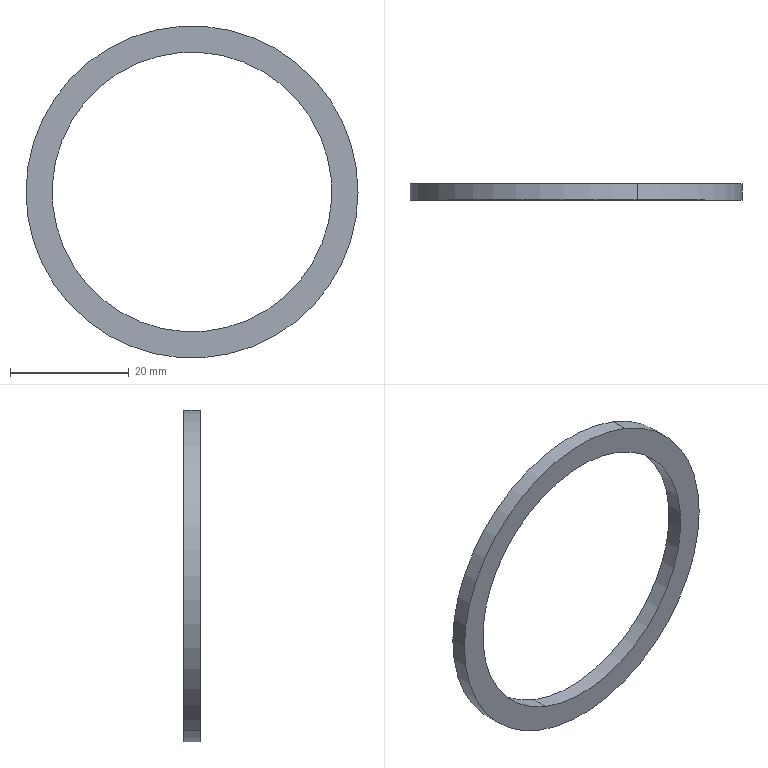Component | SolidWorks | 11-1 | 1 solid | 6 faces | box 55.8 x 2.75 x 55.8 mm | volume 1954 mm3 | cylinder 4 | plane 2 | commonest cylinder face diameters 47 x2 55.8 x2
build123d program:
from build123d import *

# Parameters (mm, degrees)
SKETCH1_R           = 27.9
SKETCH1_R_2         = 23.5
BOSS_EXTRUDE1_DEPTH = 2.75


with BuildPart() as part:
    # Sketch1 → Boss-Extrude1 (new body)
    with BuildSketch(Plane(origin=(0, 0, 0), x_dir=(1, 0, 0), z_dir=(0, 1, 0))):
        with Locations(Location((0, 0, 0), (0, 0, 270))):
            Circle(SKETCH1_R)
        with Locations(Location((0, 0, 0), (0, 0, 270))):
            Circle(SKETCH1_R_2, mode=Mode.SUBTRACT)
    extrude(amount=BOSS_EXTRUDE1_DEPTH)


solid = part.part

# Placed as in the assembly
solid = solid.moved(Location((0, -33.05, 0), (0, 0, 0)))
STEP:
#1=COLOUR_RGB('',0.7922,0.8196,0.9333);
#2=FILL_AREA_STYLE_COLOUR('',#1);
#3=FILL_AREA_STYLE('',(#2));
#4=SURFACE_STYLE_FILL_AREA(#3);
#5=SURFACE_SIDE_STYLE('',(#4));
#6=SURFACE_STYLE_USAGE(.BOTH.,#5);
#7=PRESENTATION_STYLE_ASSIGNMENT((#6));
#8=CARTESIAN_POINT('',(-0.3404,-1.193,-0.8603));
#9=VERTEX_POINT('',#8);
#10=CARTESIAN_POINT('',(0.3404,-1.193,0.8603));
#11=VERTEX_POINT('',#10);
#12=CARTESIAN_POINT('',(0.,-1.193,0.));
#13=DIRECTION('',(0.,1.,0.));
#14=DIRECTION('',(0.3679,0.,0.9299));
#15=AXIS2_PLACEMENT_3D('',#12,#13,#14);
#16=CIRCLE('',#15,0.9252);
#17=EDGE_CURVE('',#9,#11,#16,.T.);
#18=ORIENTED_EDGE('',*,*,#17,.T.);
#19=CARTESIAN_POINT('',(0.3404,-1.301,0.8603));
#20=VERTEX_POINT('',#19);
#21=CARTESIAN_POINT('',(0.3404,-1.193,0.8603));
#22=DIRECTION('',(0.,-1.,0.));
#23=VECTOR('',#22,39.37);
#24=LINE('',#21,#23);
#25=EDGE_CURVE('',#11,#20,#24,.T.);
#26=ORIENTED_EDGE('',*,*,#25,.T.);
#27=CARTESIAN_POINT('',(-0.3404,-1.301,-0.8603));
#28=VERTEX_POINT('',#27);
#29=CARTESIAN_POINT('',(0.,-1.301,0.));
#30=DIRECTION('',(0.,1.,0.));
#31=DIRECTION('',(0.3679,0.,0.9299));
#32=AXIS2_PLACEMENT_3D('',#29,#30,#31);
#33=CIRCLE('',#32,0.9252);
#34=EDGE_CURVE('',#28,#20,#33,.T.);
#35=ORIENTED_EDGE('',*,*,#34,.F.);
#36=CARTESIAN_POINT('',(-0.3404,-1.193,-0.8603));
#37=DIRECTION('',(0.,-1.,0.));
#38=VECTOR('',#37,39.37);
#39=LINE('',#36,#38);
#40=EDGE_CURVE('',#9,#28,#39,.T.);
#41=ORIENTED_EDGE('',*,*,#40,.F.);
#42=EDGE_LOOP('',(#18,#26,#35,#41));
#43=FACE_OUTER_BOUND('',#42,.T.);
#44=CARTESIAN_POINT('',(0.,-1.193,0.));
#45=DIRECTION('',(0.,-1.,0.));
#46=DIRECTION('',(-0.3679,0.,-0.9299));
#47=AXIS2_PLACEMENT_3D('',#44,#45,#46);
#48=CYLINDRICAL_SURFACE('',#47,0.9252);
#49=ADVANCED_FACE('',(#43),#48,.F.);
#50=CARTESIAN_POINT('',(0.4041,-1.193,1.021));
#51=VERTEX_POINT('',#50);
#52=CARTESIAN_POINT('',(-0.4041,-1.193,-1.021));
#53=VERTEX_POINT('',#52);
#54=CARTESIAN_POINT('',(0.,-1.193,0.));
#55=DIRECTION('',(0.,1.,0.));
#56=DIRECTION('',(0.3679,0.,0.9299));
#57=AXIS2_PLACEMENT_3D('',#54,#55,#56);
#58=CIRCLE('',#57,1.098);
#59=EDGE_CURVE('',#51,#53,#58,.T.);
#60=ORIENTED_EDGE('',*,*,#59,.F.);
#61=CARTESIAN_POINT('',(0.4041,-1.301,1.021));
#62=VERTEX_POINT('',#61);
#63=CARTESIAN_POINT('',(0.4041,-1.193,1.021));
#64=DIRECTION('',(0.,-1.,0.));
#65=VECTOR('',#64,39.37);
#66=LINE('',#63,#65);
#67=EDGE_CURVE('',#51,#62,#66,.T.);
#68=ORIENTED_EDGE('',*,*,#67,.T.);
#69=CARTESIAN_POINT('',(-0.4041,-1.301,-1.021));
#70=VERTEX_POINT('',#69);
#71=CARTESIAN_POINT('',(0.,-1.301,0.));
#72=DIRECTION('',(0.,1.,0.));
#73=DIRECTION('',(0.3679,0.,0.9299));
#74=AXIS2_PLACEMENT_3D('',#71,#72,#73);
#75=CIRCLE('',#74,1.098);
#76=EDGE_CURVE('',#62,#70,#75,.T.);
#77=ORIENTED_EDGE('',*,*,#76,.T.);
#78=CARTESIAN_POINT('',(-0.4041,-1.193,-1.021));
#79=DIRECTION('',(0.,-1.,0.));
#80=VECTOR('',#79,39.37);
#81=LINE('',#78,#80);
#82=EDGE_CURVE('',#53,#70,#81,.T.);
#83=ORIENTED_EDGE('',*,*,#82,.F.);
#84=EDGE_LOOP('',(#60,#68,#77,#83));
#85=FACE_OUTER_BOUND('',#84,.T.);
#86=CARTESIAN_POINT('',(0.,-1.193,0.));
#87=DIRECTION('',(0.,-1.,0.));
#88=DIRECTION('',(-0.3679,0.,-0.9299));
#89=AXIS2_PLACEMENT_3D('',#86,#87,#88);
#90=CYLINDRICAL_SURFACE('',#89,1.098);
#91=ADVANCED_FACE('',(#85),#90,.T.);
#92=CARTESIAN_POINT('',(0.,-1.193,0.));
#93=DIRECTION('',(0.,1.,0.));
#94=DIRECTION('',(0.3679,0.,0.9299));
#95=AXIS2_PLACEMENT_3D('',#92,#93,#94);
#96=CIRCLE('',#95,1.098);
#97=EDGE_CURVE('',#53,#51,#96,.T.);
#98=ORIENTED_EDGE('',*,*,#97,.T.);
#99=ORIENTED_EDGE('',*,*,#59,.T.);
#100=EDGE_LOOP('',(#98,#99));
#101=FACE_OUTER_BOUND('',#100,.T.);
#102=ORIENTED_EDGE('',*,*,#17,.F.);
#103=CARTESIAN_POINT('',(0.,-1.193,0.));
#104=DIRECTION('',(0.,1.,0.));
#105=DIRECTION('',(0.3679,0.,0.9299));
#106=AXIS2_PLACEMENT_3D('',#103,#104,#105);
#107=CIRCLE('',#106,0.9252);
#108=EDGE_CURVE('',#11,#9,#107,.T.);
#109=ORIENTED_EDGE('',*,*,#108,.F.);
#110=EDGE_LOOP('',(#102,#109));
#111=FACE_BOUND('',#110,.T.);
#112=CARTESIAN_POINT('',(0.,-1.193,0.));
#113=DIRECTION('',(0.,1.,0.));
#114=DIRECTION('',(0.3679,0.,0.9299));
#115=AXIS2_PLACEMENT_3D('',#112,#113,#114);
#116=PLANE('',#115);
#117=ADVANCED_FACE('',(#101,#111),#116,.T.);
#118=CARTESIAN_POINT('',(0.,-1.301,0.));
#119=DIRECTION('',(0.,1.,0.));
#120=DIRECTION('',(0.3679,0.,0.9299));
#121=AXIS2_PLACEMENT_3D('',#118,#119,#120);
#122=CIRCLE('',#121,1.098);
#123=EDGE_CURVE('',#70,#62,#122,.T.);
#124=ORIENTED_EDGE('',*,*,#123,.F.);
#125=ORIENTED_EDGE('',*,*,#76,.F.);
#126=EDGE_LOOP('',(#124,#125));
#127=FACE_OUTER_BOUND('',#126,.T.);
#128=ORIENTED_EDGE('',*,*,#34,.T.);
#129=CARTESIAN_POINT('',(0.,-1.301,0.));
#130=DIRECTION('',(0.,1.,0.));
#131=DIRECTION('',(0.3679,0.,0.9299));
#132=AXIS2_PLACEMENT_3D('',#129,#130,#131);
#133=CIRCLE('',#132,0.9252);
#134=EDGE_CURVE('',#20,#28,#133,.T.);
#135=ORIENTED_EDGE('',*,*,#134,.T.);
#136=EDGE_LOOP('',(#128,#135));
#137=FACE_BOUND('',#136,.T.);
#138=CARTESIAN_POINT('',(0.,-1.301,0.));
#139=DIRECTION('',(0.,1.,0.));
#140=DIRECTION('',(0.3679,0.,0.9299));
#141=AXIS2_PLACEMENT_3D('',#138,#139,#140);
#142=PLANE('',#141);
#143=ADVANCED_FACE('',(#127,#137),#142,.F.);
#144=ORIENTED_EDGE('',*,*,#67,.F.);
#145=ORIENTED_EDGE('',*,*,#97,.F.);
#146=ORIENTED_EDGE('',*,*,#82,.T.);
#147=ORIENTED_EDGE('',*,*,#123,.T.);
#148=EDGE_LOOP('',(#144,#145,#146,#147));
#149=FACE_OUTER_BOUND('',#148,.T.);
#150=CARTESIAN_POINT('',(0.,-1.193,0.));
#151=DIRECTION('',(0.,-1.,0.));
#152=DIRECTION('',(-0.3679,0.,-0.9299));
#153=AXIS2_PLACEMENT_3D('',#150,#151,#152);
#154=CYLINDRICAL_SURFACE('',#153,1.098);
#155=ADVANCED_FACE('',(#149),#154,.T.);
#156=ORIENTED_EDGE('',*,*,#25,.F.);
#157=ORIENTED_EDGE('',*,*,#108,.T.);
#158=ORIENTED_EDGE('',*,*,#40,.T.);
#159=ORIENTED_EDGE('',*,*,#134,.F.);
#160=EDGE_LOOP('',(#156,#157,#158,#159));
#161=FACE_OUTER_BOUND('',#160,.T.);
#162=CARTESIAN_POINT('',(0.,-1.193,0.));
#163=DIRECTION('',(0.,-1.,0.));
#164=DIRECTION('',(-0.3679,0.,-0.9299));
#165=AXIS2_PLACEMENT_3D('',#162,#163,#164);
#166=CYLINDRICAL_SURFACE('',#165,0.9252);
#167=ADVANCED_FACE('',(#161),#166,.F.);
#168=CLOSED_SHELL('',(#49,#91,#117,#143,#155,#167));
#169=MANIFOLD_SOLID_BREP('',#168);
#170=STYLED_ITEM('',(#7),#169);
#171=(LENGTH_UNIT()NAMED_UNIT(*)SI_UNIT($,.METRE.));
#172=LENGTH_MEASURE_WITH_UNIT(LENGTH_MEASURE(0.0254),#171);
#173=DIMENSIONAL_EXPONENTS(1.,0.,0.,0.,0.,0.,0.);
#174=(CONVERSION_BASED_UNIT('',#172)LENGTH_UNIT()NAMED_UNIT(#173));
#175=UNCERTAINTY_MEASURE_WITH_UNIT(LENGTH_MEASURE(0.00001),#174,'','');
#176=(NAMED_UNIT(*)PLANE_ANGLE_UNIT()SI_UNIT($,.RADIAN.));
#177=(NAMED_UNIT(*)SI_UNIT($,.STERADIAN.)SOLID_ANGLE_UNIT());
#178=(GEOMETRIC_REPRESENTATION_CONTEXT(3)GLOBAL_UNCERTAINTY_ASSIGNED_CONTEXT((#175))GLOBAL_UNIT_ASSIGNED_CONTEXT((#174,#176,#177))REPRESENTATION_CONTEXT('',''));
#179=MECHANICAL_DESIGN_GEOMETRIC_PRESENTATION_REPRESENTATION('',(#170),#178);
#180=PRESENTATION_LAYER_ASSIGNMENT('','',(#170));
#181=CARTESIAN_POINT('',(0.,0.,0.));
#182=DIRECTION('',(0.,0.,1.));
#183=DIRECTION('',(1.,0.,0.));
#184=AXIS2_PLACEMENT_3D('',#181,#182,#183);
#185=(LENGTH_UNIT()NAMED_UNIT(*)SI_UNIT($,.METRE.));
#186=LENGTH_MEASURE_WITH_UNIT(LENGTH_MEASURE(0.0254),#185);
#187=DIMENSIONAL_EXPONENTS(1.,0.,0.,0.,0.,0.,0.);
#188=(CONVERSION_BASED_UNIT('',#186)LENGTH_UNIT()NAMED_UNIT(#187));
#189=UNCERTAINTY_MEASURE_WITH_UNIT(LENGTH_MEASURE(0.00001),#188,'','');
#190=(NAMED_UNIT(*)PLANE_ANGLE_UNIT()SI_UNIT($,.RADIAN.));
#191=(NAMED_UNIT(*)SI_UNIT($,.STERADIAN.)SOLID_ANGLE_UNIT());
#192=(GEOMETRIC_REPRESENTATION_CONTEXT(3)GLOBAL_UNCERTAINTY_ASSIGNED_CONTEXT((#189))GLOBAL_UNIT_ASSIGNED_CONTEXT((#188,#190,#191))REPRESENTATION_CONTEXT('',''));
#193=ADVANCED_BREP_SHAPE_REPRESENTATION('',(#169,#184),#192);